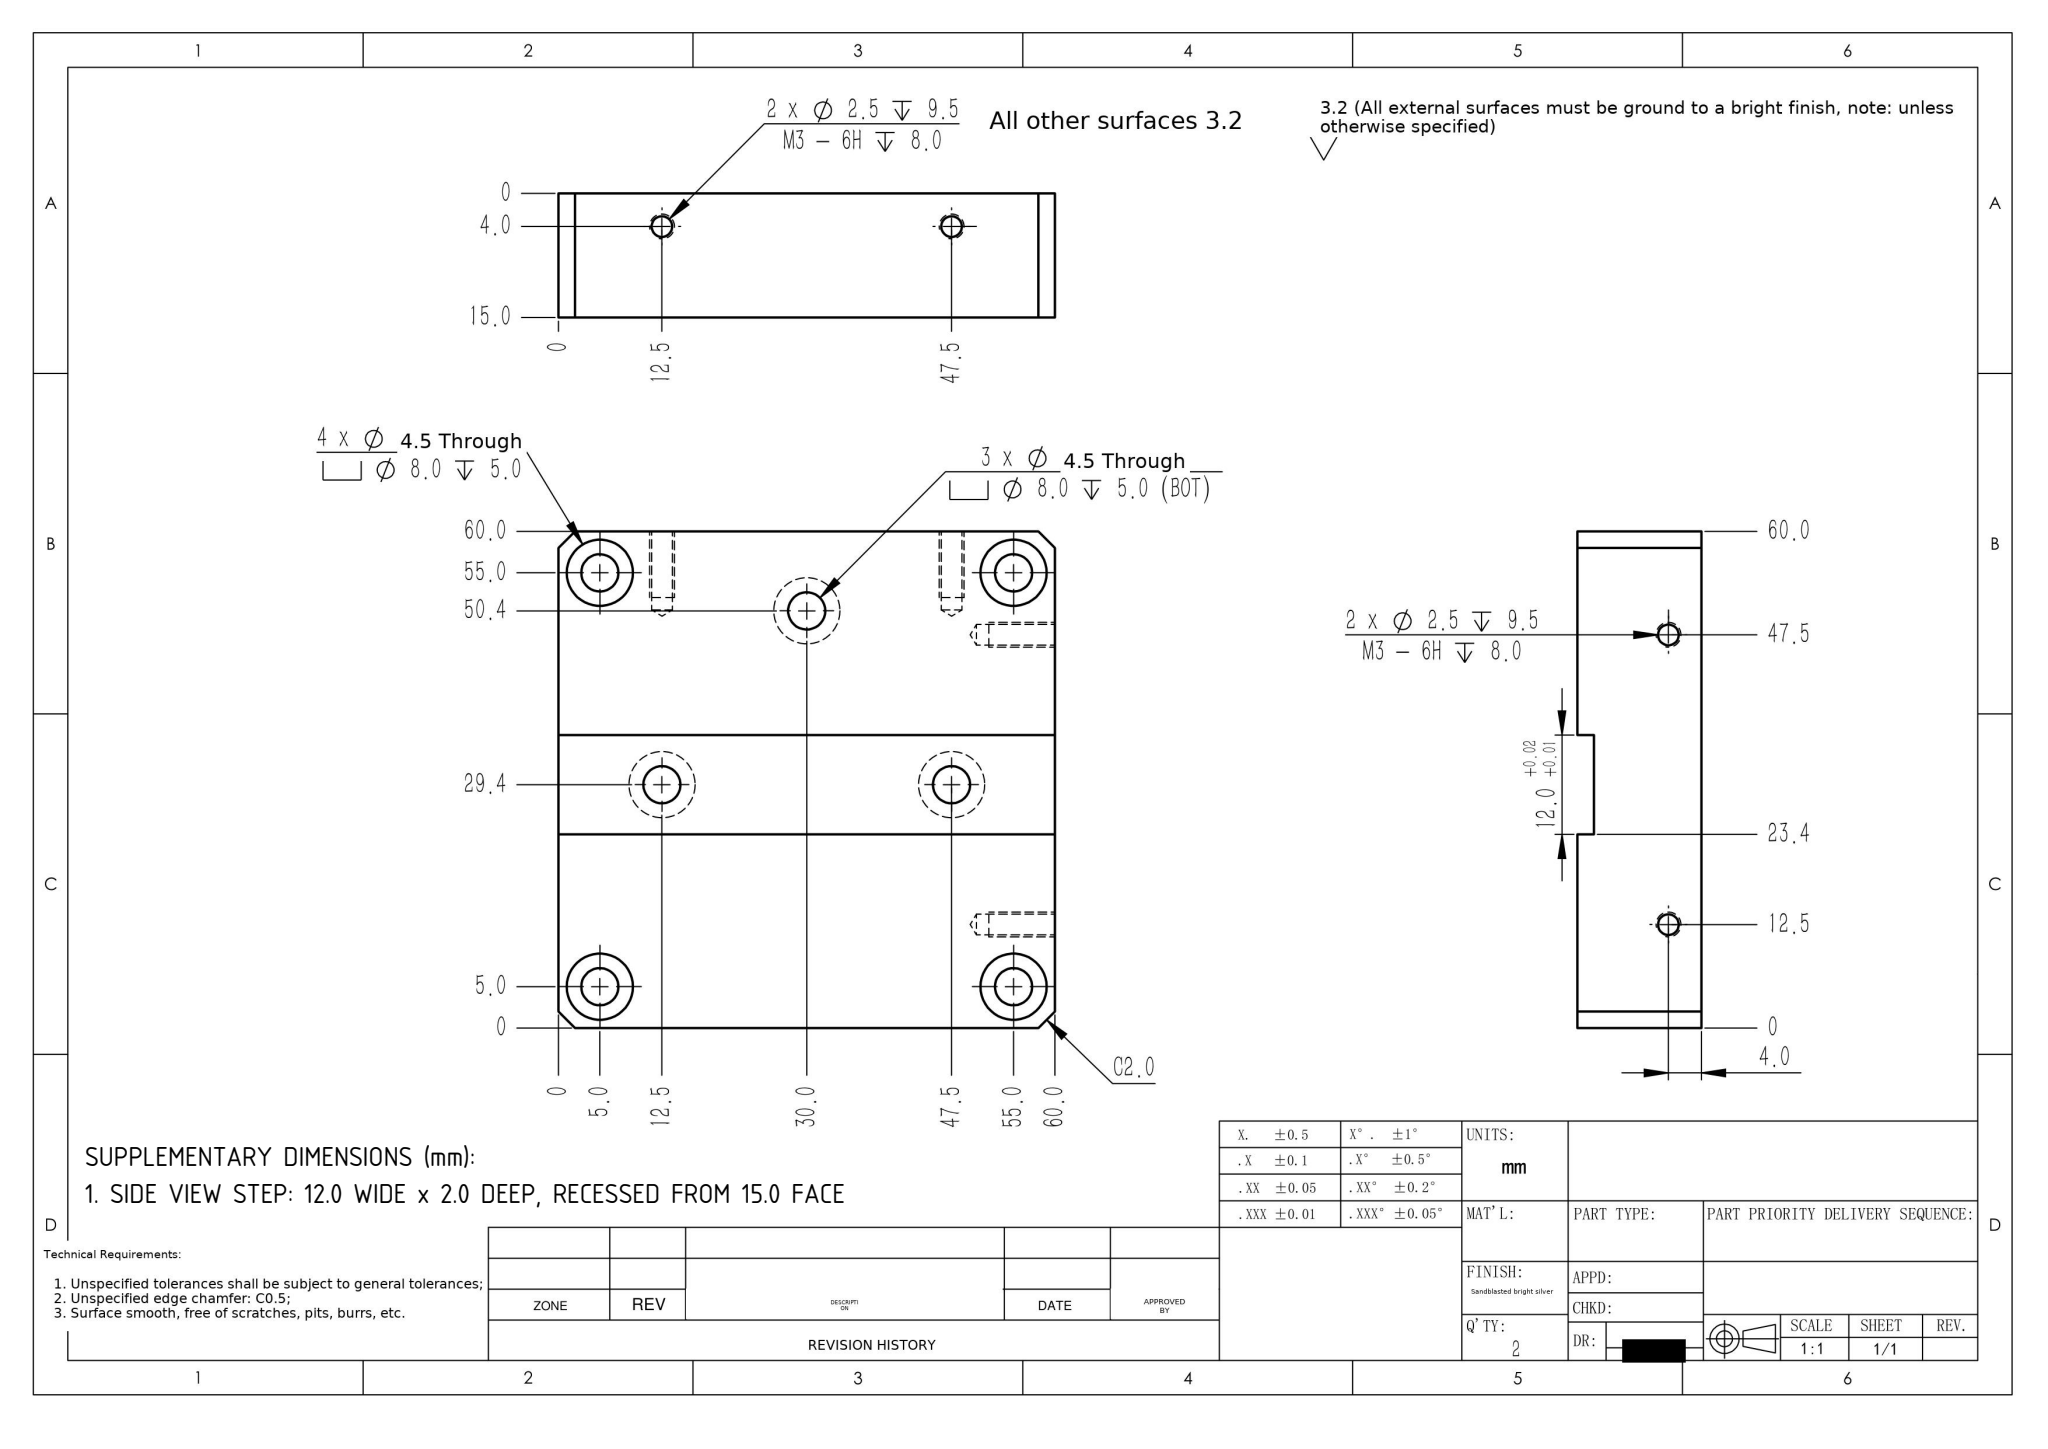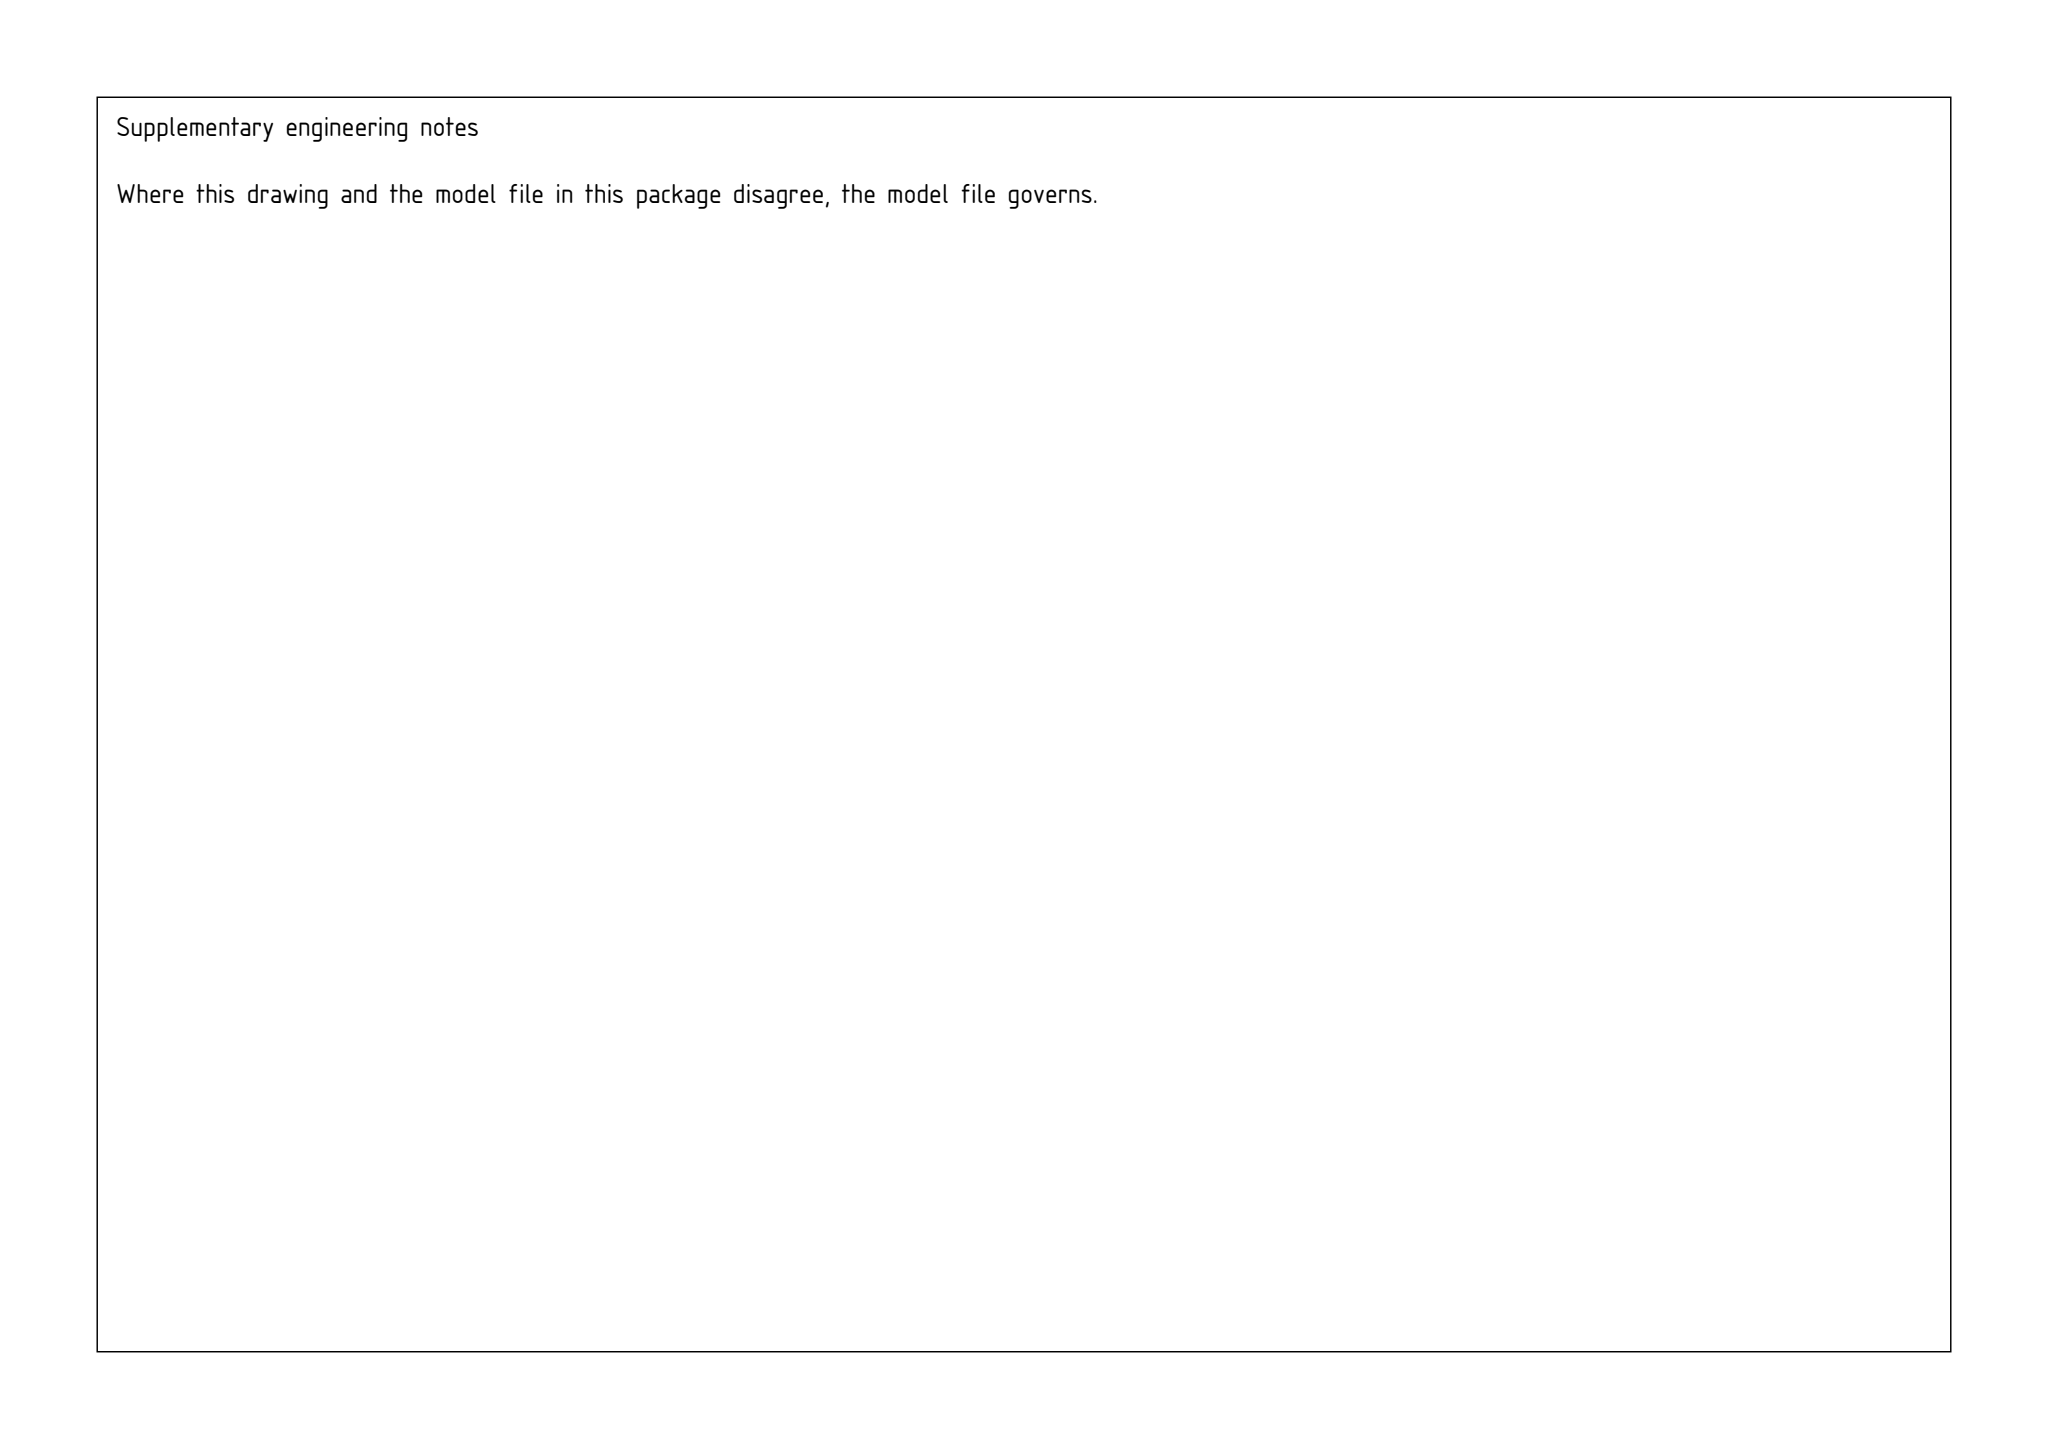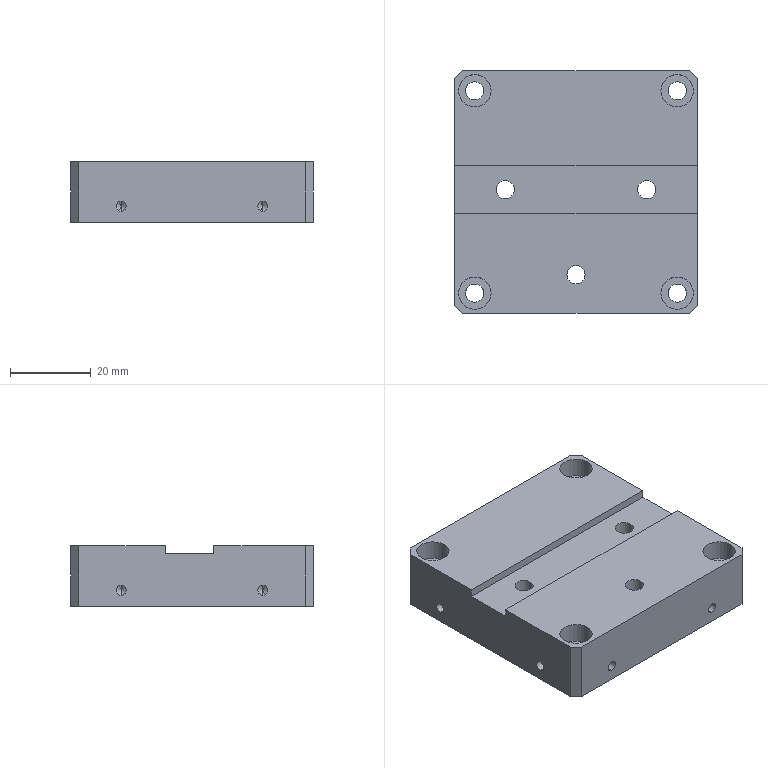Part | SolidWorks | mm | 1 solid | 65 faces | box 60 x 60 x 15 mm | volume 49440 mm3 | cylinder 36 | plane 21 | cone 8 | commonest cylinder face diameters 8 x14 4.5 x14 2.5 x8
build123d program:
from build123d import *

# Parameters (mm, degrees)
SKETCH1_W                                       = 60
SKETCH1_H                                       = 60
BOSS_EXTRUDE1_DEPTH                             = 15
M4_HEX_SOCKET_HEAD_CAP_SCREW_CBORE1_D           = 4.5
M4_HEX_SOCKET_HEAD_CAP_SCREW_CBORE1_CBORE_D     = 8
M4_HEX_SOCKET_HEAD_CAP_SCREW_CBORE1_CBORE_DEPTH = 5
SKETCH4_W                                       = 60
SKETCH4_H                                       = 12
CUT_EXTRUDE1_DEPTH                              = 2
M4_HEX_SOCKET_HEAD_CAP_SCREW_CBORE2_D           = 4.5
M4_HEX_SOCKET_HEAD_CAP_SCREW_CBORE2_CBORE_D     = 8
M4_HEX_SOCKET_HEAD_CAP_SCREW_CBORE2_CBORE_DEPTH = 5
M3_TAPPED_HOLE1_D                               = 2.5
M3_TAPPED_HOLE1_DEPTH                           = 9.5
M3_TAPPED_HOLE1_TIP                             = 0.7511
M3_TAPPED_HOLE2_D                               = 2.5
M3_TAPPED_HOLE2_DEPTH                           = 9.5
M3_TAPPED_HOLE2_TIP                             = 0.7511
CHAMFER1_SIZE                                   = 2


with BuildPart() as part:
    # Sketch1 → Boss-Extrude1 (new body)
    with BuildSketch(Plane.XY):
        Rectangle(SKETCH1_W, SKETCH1_H)
    extrude(amount=BOSS_EXTRUDE1_DEPTH)

    # M4 Hex Socket Head Cap Screw CBORE1 (through all)
    with Locations(Plane.XY.offset(15)):
        with Locations((-25, -25), (25, -25), (25, 25), (-25, 25)):
            CounterBoreHole(M4_HEX_SOCKET_HEAD_CAP_SCREW_CBORE1_D / 2, M4_HEX_SOCKET_HEAD_CAP_SCREW_CBORE1_CBORE_D / 2, M4_HEX_SOCKET_HEAD_CAP_SCREW_CBORE1_CBORE_DEPTH)

    # Sketch4 → Cut-Extrude1 (cut)
    with BuildSketch(Plane.XY.offset(15)):
        with Locations((0, 0.6)):
            Rectangle(SKETCH4_W, SKETCH4_H)
    extrude(amount=-CUT_EXTRUDE1_DEPTH, mode=Mode.SUBTRACT)

    # M4 Hex Socket Head Cap Screw CBORE2 (through all)
    with Locations(Plane(origin=(0, 0, 0), x_dir=(-1, 0, 0), z_dir=(0, 0, -1))):
        with Locations((-17.5, 0.6), (17.5, 0.6), (0, -20.4)):
            CounterBoreHole(M4_HEX_SOCKET_HEAD_CAP_SCREW_CBORE2_D / 2, M4_HEX_SOCKET_HEAD_CAP_SCREW_CBORE2_CBORE_D / 2, M4_HEX_SOCKET_HEAD_CAP_SCREW_CBORE2_CBORE_DEPTH)

    # M3 Tapped Hole1
    with Locations(Plane.ZY.offset(30)):
        with Locations((4, 17.5), (4, -17.5)):
            Hole(M3_TAPPED_HOLE1_D / 2, depth=M3_TAPPED_HOLE1_DEPTH)
            with Locations((0, 0, -(M3_TAPPED_HOLE1_DEPTH + M3_TAPPED_HOLE1_TIP / 2))):  # 118° drill point
                Cone(0, M3_TAPPED_HOLE1_D / 2, M3_TAPPED_HOLE1_TIP, mode=Mode.SUBTRACT)

    # M3 Tapped Hole2
    with Locations(Plane(origin=(0, -30, 0), x_dir=(-1, 0, 0), z_dir=(0, -1, 0))):
        with Locations((-17.5, -4), (17.5, -4)):
            Hole(M3_TAPPED_HOLE2_D / 2, depth=M3_TAPPED_HOLE2_DEPTH)
            with Locations((0, 0, -(M3_TAPPED_HOLE2_DEPTH + M3_TAPPED_HOLE2_TIP / 2))):  # 118° drill point
                Cone(0, M3_TAPPED_HOLE2_D / 2, M3_TAPPED_HOLE2_TIP, mode=Mode.SUBTRACT)

    # Chamfer1
    chamfer1_edges = [part.edges().sort_by_distance(p)[0] for p in [
        (30, -30, 7.5),
        (-30, -30, 7.5),
        (-30, 30, 7.5),
        (30, 30, 7.5),
    ]]
    chamfer(chamfer1_edges, length=CHAMFER1_SIZE)


solid = part.part